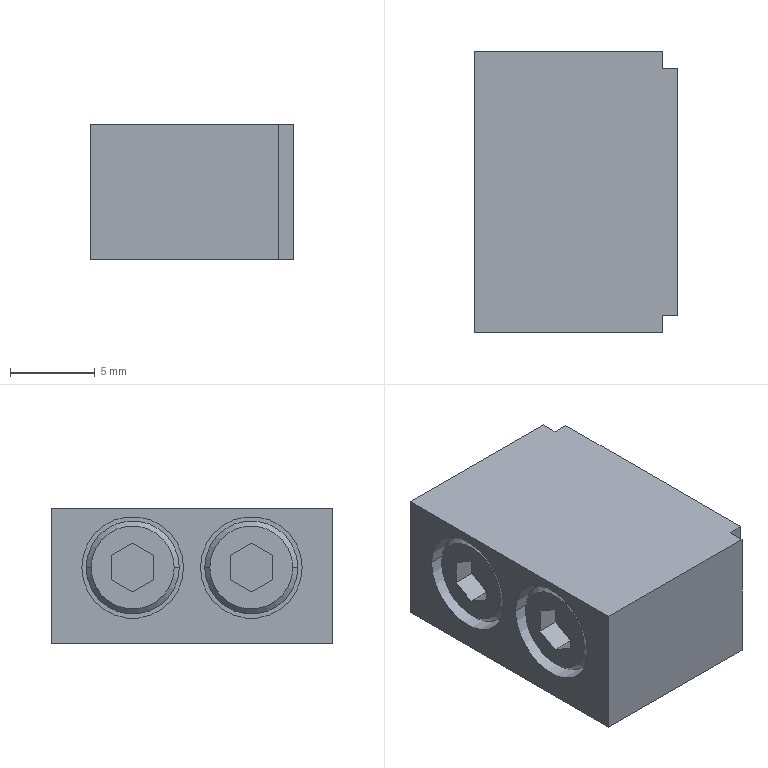Component | SolidWorks | MXQ8-30B-M9N_0_0_MXQ8-30B-M9N_0_0-2_MXQ8-30B-M9N_0_0_3_25-1 | 1 solid | 40 faces | box 12 x 16.6 x 8 mm | volume 1520 mm3 | plane 28 | cylinder 8 | cone 4 | commonest cylinder face diameters 6 x4 5.5 x4
STEP:
#1=COLOUR_RGB('',0.7922,0.8196,0.9333);
#2=FILL_AREA_STYLE_COLOUR('',#1);
#3=FILL_AREA_STYLE('',(#2));
#4=SURFACE_STYLE_FILL_AREA(#3);
#5=SURFACE_SIDE_STYLE('',(#4));
#6=SURFACE_STYLE_USAGE(.BOTH.,#5);
#7=PRESENTATION_STYLE_ASSIGNMENT((#6));
#8=CARTESIAN_POINT('',(0.7677,0.1496,1.417));
#9=VERTEX_POINT('',#8);
#10=CARTESIAN_POINT('',(0.7677,-0.08661,1.417));
#11=VERTEX_POINT('',#10);
#12=CARTESIAN_POINT('',(0.7677,0.0315,1.417));
#13=DIRECTION('',(-1.,0.,0.));
#14=DIRECTION('',(0.,-1.,0.));
#15=AXIS2_PLACEMENT_3D('',#12,#13,#14);
#16=CIRCLE('',#15,0.1181);
#17=EDGE_CURVE('',#9,#11,#16,.T.);
#18=ORIENTED_EDGE('',*,*,#17,.F.);
#19=CARTESIAN_POINT('',(0.6378,0.1496,1.417));
#20=VERTEX_POINT('',#19);
#21=CARTESIAN_POINT('',(0.6378,0.1496,1.417));
#22=DIRECTION('',(-1.,0.,0.));
#23=VECTOR('',#22,39.37);
#24=LINE('',#21,#23);
#25=EDGE_CURVE('',#9,#20,#24,.T.);
#26=ORIENTED_EDGE('',*,*,#25,.T.);
#27=CARTESIAN_POINT('',(0.6378,-0.08661,1.417));
#28=VERTEX_POINT('',#27);
#29=CARTESIAN_POINT('',(0.6378,0.0315,1.417));
#30=DIRECTION('',(1.,0.,0.));
#31=DIRECTION('',(0.,-1.,0.));
#32=AXIS2_PLACEMENT_3D('',#29,#30,#31);
#33=CIRCLE('',#32,0.1181);
#34=EDGE_CURVE('',#28,#20,#33,.T.);
#35=ORIENTED_EDGE('',*,*,#34,.F.);
#36=CARTESIAN_POINT('',(0.6378,-0.08661,1.417));
#37=DIRECTION('',(-1.,0.,0.));
#38=VECTOR('',#37,39.37);
#39=LINE('',#36,#38);
#40=EDGE_CURVE('',#11,#28,#39,.T.);
#41=ORIENTED_EDGE('',*,*,#40,.F.);
#42=EDGE_LOOP('',(#18,#26,#35,#41));
#43=FACE_OUTER_BOUND('',#42,.T.);
#44=CARTESIAN_POINT('',(0.6378,0.0315,1.417));
#45=DIRECTION('',(-1.,0.,0.));
#46=DIRECTION('',(0.,-1.,0.));
#47=AXIS2_PLACEMENT_3D('',#44,#45,#46);
#48=CYLINDRICAL_SURFACE('',#47,0.1181);
#49=ADVANCED_FACE('',(#43),#48,.F.);
#50=CARTESIAN_POINT('',(0.7677,0.4252,1.417));
#51=VERTEX_POINT('',#50);
#52=CARTESIAN_POINT('',(0.7677,0.189,1.417));
#53=VERTEX_POINT('',#52);
#54=CARTESIAN_POINT('',(0.7677,0.3071,1.417));
#55=DIRECTION('',(-1.,0.,0.));
#56=DIRECTION('',(0.,-1.,0.));
#57=AXIS2_PLACEMENT_3D('',#54,#55,#56);
#58=CIRCLE('',#57,0.1181);
#59=EDGE_CURVE('',#51,#53,#58,.T.);
#60=ORIENTED_EDGE('',*,*,#59,.F.);
#61=CARTESIAN_POINT('',(0.6378,0.4252,1.417));
#62=VERTEX_POINT('',#61);
#63=CARTESIAN_POINT('',(0.6378,0.4252,1.417));
#64=DIRECTION('',(-1.,0.,0.));
#65=VECTOR('',#64,39.37);
#66=LINE('',#63,#65);
#67=EDGE_CURVE('',#51,#62,#66,.T.);
#68=ORIENTED_EDGE('',*,*,#67,.T.);
#69=CARTESIAN_POINT('',(0.6378,0.189,1.417));
#70=VERTEX_POINT('',#69);
#71=CARTESIAN_POINT('',(0.6378,0.3071,1.417));
#72=DIRECTION('',(1.,0.,0.));
#73=DIRECTION('',(0.,-1.,0.));
#74=AXIS2_PLACEMENT_3D('',#71,#72,#73);
#75=CIRCLE('',#74,0.1181);
#76=EDGE_CURVE('',#70,#62,#75,.T.);
#77=ORIENTED_EDGE('',*,*,#76,.F.);
#78=CARTESIAN_POINT('',(0.6378,0.189,1.417));
#79=DIRECTION('',(-1.,0.,0.));
#80=VECTOR('',#79,39.37);
#81=LINE('',#78,#80);
#82=EDGE_CURVE('',#53,#70,#81,.T.);
#83=ORIENTED_EDGE('',*,*,#82,.F.);
#84=EDGE_LOOP('',(#60,#68,#77,#83));
#85=FACE_OUTER_BOUND('',#84,.T.);
#86=CARTESIAN_POINT('',(0.6378,0.3071,1.417));
#87=DIRECTION('',(-1.,0.,0.));
#88=DIRECTION('',(0.,-1.,0.));
#89=AXIS2_PLACEMENT_3D('',#86,#87,#88);
#90=CYLINDRICAL_SURFACE('',#89,0.1181);
#91=ADVANCED_FACE('',(#85),#90,.F.);
#92=CARTESIAN_POINT('',(0.6614,0.1398,1.417));
#93=VERTEX_POINT('',#92);
#94=CARTESIAN_POINT('',(0.6614,-0.07677,1.417));
#95=VERTEX_POINT('',#94);
#96=CARTESIAN_POINT('',(0.6614,0.0315,1.417));
#97=DIRECTION('',(1.,0.,0.));
#98=DIRECTION('',(0.,1.,0.));
#99=AXIS2_PLACEMENT_3D('',#96,#97,#98);
#100=CIRCLE('',#99,0.1083);
#101=EDGE_CURVE('',#93,#95,#100,.T.);
#102=ORIENTED_EDGE('',*,*,#101,.T.);
#103=CARTESIAN_POINT('',(0.7677,-0.07677,1.417));
#104=VERTEX_POINT('',#103);
#105=CARTESIAN_POINT('',(0.7146,-0.07677,1.417));
#106=DIRECTION('',(1.,0.,0.));
#107=VECTOR('',#106,39.37);
#108=LINE('',#105,#107);
#109=EDGE_CURVE('',#95,#104,#108,.T.);
#110=ORIENTED_EDGE('',*,*,#109,.T.);
#111=CARTESIAN_POINT('',(0.7677,0.1398,1.417));
#112=VERTEX_POINT('',#111);
#113=CARTESIAN_POINT('',(0.7677,0.0315,1.417));
#114=DIRECTION('',(1.,0.,0.));
#115=DIRECTION('',(0.,1.,0.));
#116=AXIS2_PLACEMENT_3D('',#113,#114,#115);
#117=CIRCLE('',#116,0.1083);
#118=EDGE_CURVE('',#112,#104,#117,.T.);
#119=ORIENTED_EDGE('',*,*,#118,.F.);
#120=CARTESIAN_POINT('',(0.7146,0.1398,1.417));
#121=DIRECTION('',(1.,0.,0.));
#122=VECTOR('',#121,39.37);
#123=LINE('',#120,#122);
#124=EDGE_CURVE('',#93,#112,#123,.T.);
#125=ORIENTED_EDGE('',*,*,#124,.F.);
#126=EDGE_LOOP('',(#102,#110,#119,#125));
#127=FACE_OUTER_BOUND('',#126,.T.);
#128=CARTESIAN_POINT('',(0.7146,0.0315,1.417));
#129=DIRECTION('',(1.,0.,0.));
#130=DIRECTION('',(0.,1.,0.));
#131=AXIS2_PLACEMENT_3D('',#128,#129,#130);
#132=CYLINDRICAL_SURFACE('',#131,0.1083);
#133=ADVANCED_FACE('',(#127),#132,.T.);
#134=CARTESIAN_POINT('',(0.6614,0.4154,1.417));
#135=VERTEX_POINT('',#134);
#136=CARTESIAN_POINT('',(0.6614,0.1988,1.417));
#137=VERTEX_POINT('',#136);
#138=CARTESIAN_POINT('',(0.6614,0.3071,1.417));
#139=DIRECTION('',(1.,0.,0.));
#140=DIRECTION('',(0.,1.,0.));
#141=AXIS2_PLACEMENT_3D('',#138,#139,#140);
#142=CIRCLE('',#141,0.1083);
#143=EDGE_CURVE('',#135,#137,#142,.T.);
#144=ORIENTED_EDGE('',*,*,#143,.T.);
#145=CARTESIAN_POINT('',(0.7677,0.1988,1.417));
#146=VERTEX_POINT('',#145);
#147=CARTESIAN_POINT('',(0.7146,0.1988,1.417));
#148=DIRECTION('',(1.,0.,0.));
#149=VECTOR('',#148,39.37);
#150=LINE('',#147,#149);
#151=EDGE_CURVE('',#137,#146,#150,.T.);
#152=ORIENTED_EDGE('',*,*,#151,.T.);
#153=CARTESIAN_POINT('',(0.7677,0.4154,1.417));
#154=VERTEX_POINT('',#153);
#155=CARTESIAN_POINT('',(0.7677,0.3071,1.417));
#156=DIRECTION('',(1.,0.,0.));
#157=DIRECTION('',(0.,1.,0.));
#158=AXIS2_PLACEMENT_3D('',#155,#156,#157);
#159=CIRCLE('',#158,0.1083);
#160=EDGE_CURVE('',#154,#146,#159,.T.);
#161=ORIENTED_EDGE('',*,*,#160,.F.);
#162=CARTESIAN_POINT('',(0.7146,0.4154,1.417));
#163=DIRECTION('',(1.,0.,0.));
#164=VECTOR('',#163,39.37);
#165=LINE('',#162,#164);
#166=EDGE_CURVE('',#135,#154,#165,.T.);
#167=ORIENTED_EDGE('',*,*,#166,.F.);
#168=EDGE_LOOP('',(#144,#152,#161,#167));
#169=FACE_OUTER_BOUND('',#168,.T.);
#170=CARTESIAN_POINT('',(0.7146,0.3071,1.417));
#171=DIRECTION('',(1.,0.,0.));
#172=DIRECTION('',(0.,1.,0.));
#173=AXIS2_PLACEMENT_3D('',#170,#171,#172);
#174=CYLINDRICAL_SURFACE('',#173,0.1083);
#175=ADVANCED_FACE('',(#169),#174,.T.);
#176=CARTESIAN_POINT('',(0.6496,0.128,1.417));
#177=VERTEX_POINT('',#176);
#178=CARTESIAN_POINT('',(0.6496,-0.06496,1.417));
#179=VERTEX_POINT('',#178);
#180=CARTESIAN_POINT('',(0.6496,0.0315,1.417));
#181=DIRECTION('',(1.,0.,0.));
#182=DIRECTION('',(0.,1.,0.));
#183=AXIS2_PLACEMENT_3D('',#180,#181,#182);
#184=CIRCLE('',#183,0.09646);
#185=EDGE_CURVE('',#177,#179,#184,.T.);
#186=ORIENTED_EDGE('',*,*,#185,.T.);
#187=CARTESIAN_POINT('',(0.6614,-0.07677,1.417));
#188=DIRECTION('',(0.7071,-0.7071,0.));
#189=VECTOR('',#188,39.37);
#190=LINE('',#187,#189);
#191=EDGE_CURVE('',#179,#95,#190,.T.);
#192=ORIENTED_EDGE('',*,*,#191,.T.);
#193=ORIENTED_EDGE('',*,*,#101,.F.);
#194=CARTESIAN_POINT('',(0.6614,0.1398,1.417));
#195=DIRECTION('',(0.7071,0.7071,0.));
#196=VECTOR('',#195,39.37);
#197=LINE('',#194,#196);
#198=EDGE_CURVE('',#177,#93,#197,.T.);
#199=ORIENTED_EDGE('',*,*,#198,.F.);
#200=EDGE_LOOP('',(#186,#192,#193,#199));
#201=FACE_OUTER_BOUND('',#200,.T.);
#202=CARTESIAN_POINT('',(0.6614,0.0315,1.417));
#203=DIRECTION('',(1.,0.,0.));
#204=DIRECTION('',(0.,1.,0.));
#205=AXIS2_PLACEMENT_3D('',#202,#203,#204);
#206=CONICAL_SURFACE('',#205,0.1083,0.7854);
#207=ADVANCED_FACE('',(#201),#206,.T.);
#208=CARTESIAN_POINT('',(0.6496,0.4035,1.417));
#209=VERTEX_POINT('',#208);
#210=CARTESIAN_POINT('',(0.6496,0.2106,1.417));
#211=VERTEX_POINT('',#210);
#212=CARTESIAN_POINT('',(0.6496,0.3071,1.417));
#213=DIRECTION('',(1.,0.,0.));
#214=DIRECTION('',(0.,1.,0.));
#215=AXIS2_PLACEMENT_3D('',#212,#213,#214);
#216=CIRCLE('',#215,0.09646);
#217=EDGE_CURVE('',#209,#211,#216,.T.);
#218=ORIENTED_EDGE('',*,*,#217,.T.);
#219=CARTESIAN_POINT('',(0.6614,0.1988,1.417));
#220=DIRECTION('',(0.7071,-0.7071,0.));
#221=VECTOR('',#220,39.37);
#222=LINE('',#219,#221);
#223=EDGE_CURVE('',#211,#137,#222,.T.);
#224=ORIENTED_EDGE('',*,*,#223,.T.);
#225=ORIENTED_EDGE('',*,*,#143,.F.);
#226=CARTESIAN_POINT('',(0.6614,0.4154,1.417));
#227=DIRECTION('',(0.7071,0.7071,0.));
#228=VECTOR('',#227,39.37);
#229=LINE('',#226,#228);
#230=EDGE_CURVE('',#209,#135,#229,.T.);
#231=ORIENTED_EDGE('',*,*,#230,.F.);
#232=EDGE_LOOP('',(#218,#224,#225,#231));
#233=FACE_OUTER_BOUND('',#232,.T.);
#234=CARTESIAN_POINT('',(0.6614,0.3071,1.417));
#235=DIRECTION('',(1.,0.,0.));
#236=DIRECTION('',(0.,1.,0.));
#237=AXIS2_PLACEMENT_3D('',#234,#235,#236);
#238=CONICAL_SURFACE('',#237,0.1083,0.7854);
#239=ADVANCED_FACE('',(#233),#238,.T.);
#240=CARTESIAN_POINT('',(0.6378,0.4961,1.555));
#241=VERTEX_POINT('',#240);
#242=CARTESIAN_POINT('',(1.075,0.4961,1.555));
#243=VERTEX_POINT('',#242);
#244=CARTESIAN_POINT('',(0.6378,0.4961,1.555));
#245=DIRECTION('',(1.,0.,0.));
#246=VECTOR('',#245,39.37);
#247=LINE('',#244,#246);
#248=EDGE_CURVE('',#241,#243,#247,.T.);
#249=ORIENTED_EDGE('',*,*,#248,.F.);
#250=CARTESIAN_POINT('',(0.6378,-0.1575,1.555));
#251=VERTEX_POINT('',#250);
#252=CARTESIAN_POINT('',(0.6378,-0.1575,1.555));
#253=DIRECTION('',(0.,1.,0.));
#254=VECTOR('',#253,39.37);
#255=LINE('',#252,#254);
#256=EDGE_CURVE('',#251,#241,#255,.T.);
#257=ORIENTED_EDGE('',*,*,#256,.F.);
#258=CARTESIAN_POINT('',(1.075,-0.1575,1.555));
#259=VERTEX_POINT('',#258);
#260=CARTESIAN_POINT('',(0.6378,-0.1575,1.555));
#261=DIRECTION('',(-1.,0.,0.));
#262=VECTOR('',#261,39.37);
#263=LINE('',#260,#262);
#264=EDGE_CURVE('',#259,#251,#263,.T.);
#265=ORIENTED_EDGE('',*,*,#264,.F.);
#266=CARTESIAN_POINT('',(1.075,-0.1181,1.555));
#267=VERTEX_POINT('',#266);
#268=CARTESIAN_POINT('',(1.075,-0.1181,1.555));
#269=DIRECTION('',(0.,1.,0.));
#270=VECTOR('',#269,39.37);
#271=LINE('',#268,#270);
#272=EDGE_CURVE('',#259,#267,#271,.T.);
#273=ORIENTED_EDGE('',*,*,#272,.T.);
#274=CARTESIAN_POINT('',(1.11,-0.1181,1.555));
#275=VERTEX_POINT('',#274);
#276=CARTESIAN_POINT('',(1.11,-0.1181,1.555));
#277=DIRECTION('',(1.,0.,0.));
#278=VECTOR('',#277,39.37);
#279=LINE('',#276,#278);
#280=EDGE_CURVE('',#267,#275,#279,.T.);
#281=ORIENTED_EDGE('',*,*,#280,.T.);
#282=CARTESIAN_POINT('',(1.11,0.4567,1.555));
#283=VERTEX_POINT('',#282);
#284=CARTESIAN_POINT('',(1.11,-0.1575,1.555));
#285=DIRECTION('',(0.,-1.,0.));
#286=VECTOR('',#285,39.37);
#287=LINE('',#284,#286);
#288=EDGE_CURVE('',#283,#275,#287,.T.);
#289=ORIENTED_EDGE('',*,*,#288,.F.);
#290=CARTESIAN_POINT('',(1.075,0.4567,1.555));
#291=VERTEX_POINT('',#290);
#292=CARTESIAN_POINT('',(1.075,0.4567,1.555));
#293=DIRECTION('',(-1.,0.,0.));
#294=VECTOR('',#293,39.37);
#295=LINE('',#292,#294);
#296=EDGE_CURVE('',#283,#291,#295,.T.);
#297=ORIENTED_EDGE('',*,*,#296,.T.);
#298=CARTESIAN_POINT('',(1.075,0.4961,1.555));
#299=DIRECTION('',(0.,1.,0.));
#300=VECTOR('',#299,39.37);
#301=LINE('',#298,#300);
#302=EDGE_CURVE('',#291,#243,#301,.T.);
#303=ORIENTED_EDGE('',*,*,#302,.T.);
#304=EDGE_LOOP('',(#249,#257,#265,#273,#281,#289,#297,#303));
#305=FACE_OUTER_BOUND('',#304,.T.);
#306=CARTESIAN_POINT('',(0.6378,-0.1575,1.555));
#307=DIRECTION('',(0.,0.,-1.));
#308=DIRECTION('',(0.,1.,0.));
#309=AXIS2_PLACEMENT_3D('',#306,#307,#308);
#310=PLANE('',#309);
#311=ADVANCED_FACE('',(#305),#310,.F.);
#312=CARTESIAN_POINT('',(0.6378,0.4961,1.24));
#313=VERTEX_POINT('',#312);
#314=CARTESIAN_POINT('',(0.6378,0.4961,1.555));
#315=DIRECTION('',(0.,0.,1.));
#316=VECTOR('',#315,39.37);
#317=LINE('',#314,#316);
#318=EDGE_CURVE('',#313,#241,#317,.T.);
#319=ORIENTED_EDGE('',*,*,#318,.T.);
#320=ORIENTED_EDGE('',*,*,#248,.T.);
#321=CARTESIAN_POINT('',(1.075,0.4961,1.24));
#322=VERTEX_POINT('',#321);
#323=CARTESIAN_POINT('',(1.075,0.4961,1.555));
#324=DIRECTION('',(0.,0.,-1.));
#325=VECTOR('',#324,39.37);
#326=LINE('',#323,#325);
#327=EDGE_CURVE('',#243,#322,#326,.T.);
#328=ORIENTED_EDGE('',*,*,#327,.T.);
#329=CARTESIAN_POINT('',(1.11,0.4961,1.24));
#330=DIRECTION('',(-1.,0.,0.));
#331=VECTOR('',#330,39.37);
#332=LINE('',#329,#331);
#333=EDGE_CURVE('',#322,#313,#332,.T.);
#334=ORIENTED_EDGE('',*,*,#333,.T.);
#335=EDGE_LOOP('',(#319,#320,#328,#334));
#336=FACE_OUTER_BOUND('',#335,.T.);
#337=CARTESIAN_POINT('',(1.11,0.4961,1.555));
#338=DIRECTION('',(0.,1.,0.));
#339=DIRECTION('',(-1.,0.,0.));
#340=AXIS2_PLACEMENT_3D('',#337,#338,#339);
#341=PLANE('',#340);
#342=ADVANCED_FACE('',(#336),#341,.T.);
#343=ORIENTED_EDGE('',*,*,#256,.T.);
#344=ORIENTED_EDGE('',*,*,#318,.F.);
#345=CARTESIAN_POINT('',(0.6378,-0.1575,1.24));
#346=VERTEX_POINT('',#345);
#347=CARTESIAN_POINT('',(0.6378,0.4961,1.24));
#348=DIRECTION('',(0.,-1.,0.));
#349=VECTOR('',#348,39.37);
#350=LINE('',#347,#349);
#351=EDGE_CURVE('',#313,#346,#350,.T.);
#352=ORIENTED_EDGE('',*,*,#351,.T.);
#353=CARTESIAN_POINT('',(0.6378,-0.1575,1.555));
#354=DIRECTION('',(0.,0.,1.));
#355=VECTOR('',#354,39.37);
#356=LINE('',#353,#355);
#357=EDGE_CURVE('',#346,#251,#356,.T.);
#358=ORIENTED_EDGE('',*,*,#357,.T.);
#359=EDGE_LOOP('',(#343,#344,#352,#358));
#360=FACE_OUTER_BOUND('',#359,.T.);
#361=ORIENTED_EDGE('',*,*,#34,.T.);
#362=CARTESIAN_POINT('',(0.6378,0.0315,1.417));
#363=DIRECTION('',(1.,0.,0.));
#364=DIRECTION('',(0.,-1.,0.));
#365=AXIS2_PLACEMENT_3D('',#362,#363,#364);
#366=CIRCLE('',#365,0.1181);
#367=EDGE_CURVE('',#20,#28,#366,.T.);
#368=ORIENTED_EDGE('',*,*,#367,.T.);
#369=EDGE_LOOP('',(#361,#368));
#370=FACE_BOUND('',#369,.T.);
#371=ORIENTED_EDGE('',*,*,#76,.T.);
#372=CARTESIAN_POINT('',(0.6378,0.3071,1.417));
#373=DIRECTION('',(1.,0.,0.));
#374=DIRECTION('',(0.,-1.,0.));
#375=AXIS2_PLACEMENT_3D('',#372,#373,#374);
#376=CIRCLE('',#375,0.1181);
#377=EDGE_CURVE('',#62,#70,#376,.T.);
#378=ORIENTED_EDGE('',*,*,#377,.T.);
#379=EDGE_LOOP('',(#371,#378));
#380=FACE_BOUND('',#379,.T.);
#381=CARTESIAN_POINT('',(0.6378,0.4961,1.555));
#382=DIRECTION('',(-1.,0.,0.));
#383=DIRECTION('',(0.,-1.,0.));
#384=AXIS2_PLACEMENT_3D('',#381,#382,#383);
#385=PLANE('',#384);
#386=ADVANCED_FACE('',(#360,#370,#380),#385,.T.);
#387=ORIENTED_EDGE('',*,*,#357,.F.);
#388=CARTESIAN_POINT('',(1.075,-0.1575,1.24));
#389=VERTEX_POINT('',#388);
#390=CARTESIAN_POINT('',(0.6378,-0.1575,1.24));
#391=DIRECTION('',(1.,0.,0.));
#392=VECTOR('',#391,39.37);
#393=LINE('',#390,#392);
#394=EDGE_CURVE('',#346,#389,#393,.T.);
#395=ORIENTED_EDGE('',*,*,#394,.T.);
#396=CARTESIAN_POINT('',(1.075,-0.1575,1.555));
#397=DIRECTION('',(0.,0.,1.));
#398=VECTOR('',#397,39.37);
#399=LINE('',#396,#398);
#400=EDGE_CURVE('',#389,#259,#399,.T.);
#401=ORIENTED_EDGE('',*,*,#400,.T.);
#402=ORIENTED_EDGE('',*,*,#264,.T.);
#403=EDGE_LOOP('',(#387,#395,#401,#402));
#404=FACE_OUTER_BOUND('',#403,.T.);
#405=CARTESIAN_POINT('',(0.6378,-0.1575,1.555));
#406=DIRECTION('',(0.,-1.,0.));
#407=DIRECTION('',(1.,0.,0.));
#408=AXIS2_PLACEMENT_3D('',#405,#406,#407);
#409=PLANE('',#408);
#410=ADVANCED_FACE('',(#404),#409,.T.);
#411=CARTESIAN_POINT('',(1.11,-0.1181,1.24));
#412=VERTEX_POINT('',#411);
#413=CARTESIAN_POINT('',(1.11,-0.1181,1.555));
#414=DIRECTION('',(0.,0.,-1.));
#415=VECTOR('',#414,39.37);
#416=LINE('',#413,#415);
#417=EDGE_CURVE('',#275,#412,#416,.T.);
#418=ORIENTED_EDGE('',*,*,#417,.T.);
#419=CARTESIAN_POINT('',(1.11,0.4567,1.24));
#420=VERTEX_POINT('',#419);
#421=CARTESIAN_POINT('',(1.11,-0.1575,1.24));
#422=DIRECTION('',(0.,1.,0.));
#423=VECTOR('',#422,39.37);
#424=LINE('',#421,#423);
#425=EDGE_CURVE('',#412,#420,#424,.T.);
#426=ORIENTED_EDGE('',*,*,#425,.T.);
#427=CARTESIAN_POINT('',(1.11,0.4567,1.555));
#428=DIRECTION('',(0.,0.,1.));
#429=VECTOR('',#428,39.37);
#430=LINE('',#427,#429);
#431=EDGE_CURVE('',#420,#283,#430,.T.);
#432=ORIENTED_EDGE('',*,*,#431,.T.);
#433=ORIENTED_EDGE('',*,*,#288,.T.);
#434=EDGE_LOOP('',(#418,#426,#432,#433));
#435=FACE_OUTER_BOUND('',#434,.T.);
#436=CARTESIAN_POINT('',(1.11,-0.1575,1.555));
#437=DIRECTION('',(1.,0.,0.));
#438=DIRECTION('',(0.,1.,0.));
#439=AXIS2_PLACEMENT_3D('',#436,#437,#438);
#440=PLANE('',#439);
#441=ADVANCED_FACE('',(#435),#440,.T.);
#442=ORIENTED_EDGE('',*,*,#351,.F.);
#443=ORIENTED_EDGE('',*,*,#333,.F.);
#444=CARTESIAN_POINT('',(1.075,0.4567,1.24));
#445=VERTEX_POINT('',#444);
#446=CARTESIAN_POINT('',(1.075,-0.1575,1.24));
#447=DIRECTION('',(0.,-1.,0.));
#448=VECTOR('',#447,39.37);
#449=LINE('',#446,#448);
#450=EDGE_CURVE('',#322,#445,#449,.T.);
#451=ORIENTED_EDGE('',*,*,#450,.T.);
#452=CARTESIAN_POINT('',(0.6378,0.4567,1.24));
#453=DIRECTION('',(1.,0.,0.));
#454=VECTOR('',#453,39.37);
#455=LINE('',#452,#454);
#456=EDGE_CURVE('',#445,#420,#455,.T.);
#457=ORIENTED_EDGE('',*,*,#456,.T.);
#458=ORIENTED_EDGE('',*,*,#425,.F.);
#459=CARTESIAN_POINT('',(1.075,-0.1181,1.24));
#460=VERTEX_POINT('',#459);
#461=CARTESIAN_POINT('',(0.6378,-0.1181,1.24));
#462=DIRECTION('',(-1.,0.,0.));
#463=VECTOR('',#462,39.37);
#464=LINE('',#461,#463);
#465=EDGE_CURVE('',#412,#460,#464,.T.);
#466=ORIENTED_EDGE('',*,*,#465,.T.);
#467=CARTESIAN_POINT('',(1.075,-0.1575,1.24));
#468=DIRECTION('',(0.,-1.,0.));
#469=VECTOR('',#468,39.37);
#470=LINE('',#467,#469);
#471=EDGE_CURVE('',#460,#389,#470,.T.);
#472=ORIENTED_EDGE('',*,*,#471,.T.);
#473=ORIENTED_EDGE('',*,*,#394,.F.);
#474=EDGE_LOOP('',(#442,#443,#451,#457,#458,#466,#472,#473));
#475=FACE_OUTER_BOUND('',#474,.T.);
#476=CARTESIAN_POINT('',(0.6378,-0.1575,1.24));
#477=DIRECTION('',(0.,0.,-1.));
#478=DIRECTION('',(0.,1.,0.));
#479=AXIS2_PLACEMENT_3D('',#476,#477,#478);
#480=PLANE('',#479);
#481=ADVANCED_FACE('',(#475),#480,.T.);
#482=ORIENTED_EDGE('',*,*,#327,.F.);
#483=ORIENTED_EDGE('',*,*,#302,.F.);
#484=CARTESIAN_POINT('',(1.075,0.4567,1.555));
#485=DIRECTION('',(0.,0.,1.));
#486=VECTOR('',#485,39.37);
#487=LINE('',#484,#486);
#488=EDGE_CURVE('',#445,#291,#487,.T.);
#489=ORIENTED_EDGE('',*,*,#488,.F.);
#490=ORIENTED_EDGE('',*,*,#450,.F.);
#491=EDGE_LOOP('',(#482,#483,#489,#490));
#492=FACE_OUTER_BOUND('',#491,.T.);
#493=CARTESIAN_POINT('',(1.075,0.4961,1.555));
#494=DIRECTION('',(-1.,0.,0.));
#495=DIRECTION('',(0.,-1.,0.));
#496=AXIS2_PLACEMENT_3D('',#493,#494,#495);
#497=PLANE('',#496);
#498=ADVANCED_FACE('',(#492),#497,.F.);
#499=ORIENTED_EDGE('',*,*,#25,.F.);
#500=CARTESIAN_POINT('',(0.7677,0.0315,1.417));
#501=DIRECTION('',(-1.,0.,0.));
#502=DIRECTION('',(0.,-1.,0.));
#503=AXIS2_PLACEMENT_3D('',#500,#501,#502);
#504=CIRCLE('',#503,0.1181);
#505=EDGE_CURVE('',#11,#9,#504,.T.);
#506=ORIENTED_EDGE('',*,*,#505,.F.);
#507=ORIENTED_EDGE('',*,*,#40,.T.);
#508=ORIENTED_EDGE('',*,*,#367,.F.);
#509=EDGE_LOOP('',(#499,#506,#507,#508));
#510=FACE_OUTER_BOUND('',#509,.T.);
#511=CARTESIAN_POINT('',(0.6378,0.0315,1.417));
#512=DIRECTION('',(-1.,0.,0.));
#513=DIRECTION('',(0.,-1.,0.));
#514=AXIS2_PLACEMENT_3D('',#511,#512,#513);
#515=CYLINDRICAL_SURFACE('',#514,0.1181);
#516=ADVANCED_FACE('',(#510),#515,.F.);
#517=ORIENTED_EDGE('',*,*,#67,.F.);
#518=CARTESIAN_POINT('',(0.7677,0.3071,1.417));
#519=DIRECTION('',(-1.,0.,0.));
#520=DIRECTION('',(0.,-1.,0.));
#521=AXIS2_PLACEMENT_3D('',#518,#519,#520);
#522=CIRCLE('',#521,0.1181);
#523=EDGE_CURVE('',#53,#51,#522,.T.);
#524=ORIENTED_EDGE('',*,*,#523,.F.);
#525=ORIENTED_EDGE('',*,*,#82,.T.);
#526=ORIENTED_EDGE('',*,*,#377,.F.);
#527=EDGE_LOOP('',(#517,#524,#525,#526));
#528=FACE_OUTER_BOUND('',#527,.T.);
#529=CARTESIAN_POINT('',(0.6378,0.3071,1.417));
#530=DIRECTION('',(-1.,0.,0.));
#531=DIRECTION('',(0.,-1.,0.));
#532=AXIS2_PLACEMENT_3D('',#529,#530,#531);
#533=CYLINDRICAL_SURFACE('',#532,0.1181);
#534=ADVANCED_FACE('',(#528),#533,.F.);
#535=CARTESIAN_POINT('',(1.075,-0.1181,1.555));
#536=DIRECTION('',(0.,0.,-1.));
#537=VECTOR('',#536,39.37);
#538=LINE('',#535,#537);
#539=EDGE_CURVE('',#267,#460,#538,.T.);
#540=ORIENTED_EDGE('',*,*,#539,.F.);
#541=ORIENTED_EDGE('',*,*,#272,.F.);
#542=ORIENTED_EDGE('',*,*,#400,.F.);
#543=ORIENTED_EDGE('',*,*,#471,.F.);
#544=EDGE_LOOP('',(#540,#541,#542,#543));
#545=FACE_OUTER_BOUND('',#544,.T.);
#546=CARTESIAN_POINT('',(1.075,-0.1181,1.555));
#547=DIRECTION('',(-1.,0.,0.));
#548=DIRECTION('',(0.,-1.,0.));
#549=AXIS2_PLACEMENT_3D('',#546,#547,#548);
#550=PLANE('',#549);
#551=ADVANCED_FACE('',(#545),#550,.F.);
#552=ORIENTED_EDGE('',*,*,#417,.F.);
#553=ORIENTED_EDGE('',*,*,#280,.F.);
#554=ORIENTED_EDGE('',*,*,#539,.T.);
#555=ORIENTED_EDGE('',*,*,#465,.F.);
#556=EDGE_LOOP('',(#552,#553,#554,#555));
#557=FACE_OUTER_BOUND('',#556,.T.);
#558=CARTESIAN_POINT('',(1.11,-0.1181,1.555));
#559=DIRECTION('',(0.,1.,0.));
#560=DIRECTION('',(-1.,0.,0.));
#561=AXIS2_PLACEMENT_3D('',#558,#559,#560);
#562=PLANE('',#561);
#563=ADVANCED_FACE('',(#557),#562,.F.);
#564=ORIENTED_EDGE('',*,*,#488,.T.);
#565=ORIENTED_EDGE('',*,*,#296,.F.);
#566=ORIENTED_EDGE('',*,*,#431,.F.);
#567=ORIENTED_EDGE('',*,*,#456,.F.);
#568=EDGE_LOOP('',(#564,#565,#566,#567));
#569=FACE_OUTER_BOUND('',#568,.T.);
#570=CARTESIAN_POINT('',(1.075,0.4567,1.555));
#571=DIRECTION('',(0.,-1.,0.));
#572=DIRECTION('',(1.,0.,0.));
#573=AXIS2_PLACEMENT_3D('',#570,#571,#572);
#574=PLANE('',#573);
#575=ADVANCED_FACE('',(#569),#574,.F.);
#576=ORIENTED_EDGE('',*,*,#505,.T.);
#577=ORIENTED_EDGE('',*,*,#17,.T.);
#578=EDGE_LOOP('',(#576,#577));
#579=FACE_OUTER_BOUND('',#578,.T.);
#580=ORIENTED_EDGE('',*,*,#118,.T.);
#581=CARTESIAN_POINT('',(0.7677,0.0315,1.417));
#582=DIRECTION('',(1.,0.,0.));
#583=DIRECTION('',(0.,1.,0.));
#584=AXIS2_PLACEMENT_3D('',#581,#582,#583);
#585=CIRCLE('',#584,0.1083);
#586=EDGE_CURVE('',#104,#112,#585,.T.);
#587=ORIENTED_EDGE('',*,*,#586,.T.);
#588=EDGE_LOOP('',(#580,#587));
#589=FACE_BOUND('',#588,.T.);
#590=CARTESIAN_POINT('',(0.7677,-0.1575,1.555));
#591=DIRECTION('',(-1.,0.,0.));
#592=DIRECTION('',(0.,-1.,0.));
#593=AXIS2_PLACEMENT_3D('',#590,#591,#592);
#594=PLANE('',#593);
#595=ADVANCED_FACE('',(#579,#589),#594,.T.);
#596=ORIENTED_EDGE('',*,*,#523,.T.);
#597=ORIENTED_EDGE('',*,*,#59,.T.);
#598=EDGE_LOOP('',(#596,#597));
#599=FACE_OUTER_BOUND('',#598,.T.);
#600=ORIENTED_EDGE('',*,*,#160,.T.);
#601=CARTESIAN_POINT('',(0.7677,0.3071,1.417));
#602=DIRECTION('',(1.,0.,0.));
#603=DIRECTION('',(0.,1.,0.));
#604=AXIS2_PLACEMENT_3D('',#601,#602,#603);
#605=CIRCLE('',#604,0.1083);
#606=EDGE_CURVE('',#146,#154,#605,.T.);
#607=ORIENTED_EDGE('',*,*,#606,.T.);
#608=EDGE_LOOP('',(#600,#607));
#609=FACE_BOUND('',#608,.T.);
#610=CARTESIAN_POINT('',(0.7677,-0.1575,1.555));
#611=DIRECTION('',(-1.,0.,0.));
#612=DIRECTION('',(0.,-1.,0.));
#613=AXIS2_PLACEMENT_3D('',#610,#611,#612);
#614=PLANE('',#613);
#615=ADVANCED_FACE('',(#599,#609),#614,.T.);
#616=ORIENTED_EDGE('',*,*,#109,.F.);
#617=CARTESIAN_POINT('',(0.6614,0.0315,1.417));
#618=DIRECTION('',(1.,0.,0.));
#619=DIRECTION('',(0.,1.,0.));
#620=AXIS2_PLACEMENT_3D('',#617,#618,#619);
#621=CIRCLE('',#620,0.1083);
#622=EDGE_CURVE('',#95,#93,#621,.T.);
#623=ORIENTED_EDGE('',*,*,#622,.T.);
#624=ORIENTED_EDGE('',*,*,#124,.T.);
#625=ORIENTED_EDGE('',*,*,#586,.F.);
#626=EDGE_LOOP('',(#616,#623,#624,#625));
#627=FACE_OUTER_BOUND('',#626,.T.);
#628=CARTESIAN_POINT('',(0.7146,0.0315,1.417));
#629=DIRECTION('',(1.,0.,0.));
#630=DIRECTION('',(0.,1.,0.));
#631=AXIS2_PLACEMENT_3D('',#628,#629,#630);
#632=CYLINDRICAL_SURFACE('',#631,0.1083);
#633=ADVANCED_FACE('',(#627),#632,.T.);
#634=ORIENTED_EDGE('',*,*,#151,.F.);
#635=CARTESIAN_POINT('',(0.6614,0.3071,1.417));
#636=DIRECTION('',(1.,0.,0.));
#637=DIRECTION('',(0.,1.,0.));
#638=AXIS2_PLACEMENT_3D('',#635,#636,#637);
#639=CIRCLE('',#638,0.1083);
#640=EDGE_CURVE('',#137,#135,#639,.T.);
#641=ORIENTED_EDGE('',*,*,#640,.T.);
#642=ORIENTED_EDGE('',*,*,#166,.T.);
#643=ORIENTED_EDGE('',*,*,#606,.F.);
#644=EDGE_LOOP('',(#634,#641,#642,#643));
#645=FACE_OUTER_BOUND('',#644,.T.);
#646=CARTESIAN_POINT('',(0.7146,0.3071,1.417));
#647=DIRECTION('',(1.,0.,0.));
#648=DIRECTION('',(0.,1.,0.));
#649=AXIS2_PLACEMENT_3D('',#646,#647,#648);
#650=CYLINDRICAL_SURFACE('',#649,0.1083);
#651=ADVANCED_FACE('',(#645),#650,.T.);
#652=ORIENTED_EDGE('',*,*,#191,.F.);
#653=CARTESIAN_POINT('',(0.6496,0.0315,1.417));
#654=DIRECTION('',(1.,0.,0.));
#655=DIRECTION('',(0.,1.,0.));
#656=AXIS2_PLACEMENT_3D('',#653,#654,#655);
#657=CIRCLE('',#656,0.09646);
#658=EDGE_CURVE('',#179,#177,#657,.T.);
#659=ORIENTED_EDGE('',*,*,#658,.T.);
#660=ORIENTED_EDGE('',*,*,#198,.T.);
#661=ORIENTED_EDGE('',*,*,#622,.F.);
#662=EDGE_LOOP('',(#652,#659,#660,#661));
#663=FACE_OUTER_BOUND('',#662,.T.);
#664=CARTESIAN_POINT('',(0.6614,0.0315,1.417));
#665=DIRECTION('',(1.,0.,0.));
#666=DIRECTION('',(0.,1.,0.));
#667=AXIS2_PLACEMENT_3D('',#664,#665,#666);
#668=CONICAL_SURFACE('',#667,0.1083,0.7854);
#669=ADVANCED_FACE('',(#663),#668,.T.);
#670=ORIENTED_EDGE('',*,*,#223,.F.);
#671=CARTESIAN_POINT('',(0.6496,0.3071,1.417));
#672=DIRECTION('',(1.,0.,0.));
#673=DIRECTION('',(0.,1.,0.));
#674=AXIS2_PLACEMENT_3D('',#671,#672,#673);
#675=CIRCLE('',#674,0.09646);
#676=EDGE_CURVE('',#211,#209,#675,.T.);
#677=ORIENTED_EDGE('',*,*,#676,.T.);
#678=ORIENTED_EDGE('',*,*,#230,.T.);
#679=ORIENTED_EDGE('',*,*,#640,.F.);
#680=EDGE_LOOP('',(#670,#677,#678,#679));
#681=FACE_OUTER_BOUND('',#680,.T.);
#682=CARTESIAN_POINT('',(0.6614,0.3071,1.417));
#683=DIRECTION('',(1.,0.,0.));
#684=DIRECTION('',(0.,1.,0.));
#685=AXIS2_PLACEMENT_3D('',#682,#683,#684);
#686=CONICAL_SURFACE('',#685,0.1083,0.7854);
#687=ADVANCED_FACE('',(#681),#686,.T.);
#688=ORIENTED_EDGE('',*,*,#185,.F.);
#689=ORIENTED_EDGE('',*,*,#658,.F.);
#690=EDGE_LOOP('',(#688,#689));
#691=FACE_OUTER_BOUND('',#690,.T.);
#692=CARTESIAN_POINT('',(0.6496,0.0315,1.36));
#693=VERTEX_POINT('',#692);
#694=CARTESIAN_POINT('',(0.6496,0.08071,1.389));
#695=VERTEX_POINT('',#694);
#696=CARTESIAN_POINT('',(0.6496,0.0315,1.36));
#697=DIRECTION('',(0.,0.866,0.5));
#698=VECTOR('',#697,39.37);
#699=LINE('',#696,#698);
#700=EDGE_CURVE('',#693,#695,#699,.T.);
#701=ORIENTED_EDGE('',*,*,#700,.T.);
#702=CARTESIAN_POINT('',(0.6496,0.08071,1.446));
#703=VERTEX_POINT('',#702);
#704=CARTESIAN_POINT('',(0.6496,0.08071,1.369));
#705=DIRECTION('',(0.,0.,1.));
#706=VECTOR('',#705,39.37);
#707=LINE('',#704,#706);
#708=EDGE_CURVE('',#695,#703,#707,.T.);
#709=ORIENTED_EDGE('',*,*,#708,.T.);
#710=CARTESIAN_POINT('',(0.6496,0.0315,1.474));
#711=VERTEX_POINT('',#710);
#712=CARTESIAN_POINT('',(0.6496,0.08071,1.446));
#713=DIRECTION('',(0.,-0.866,0.5));
#714=VECTOR('',#713,39.37);
#715=LINE('',#712,#714);
#716=EDGE_CURVE('',#703,#711,#715,.T.);
#717=ORIENTED_EDGE('',*,*,#716,.T.);
#718=CARTESIAN_POINT('',(0.6496,-0.01772,1.446));
#719=VERTEX_POINT('',#718);
#720=CARTESIAN_POINT('',(0.6496,0.0315,1.474));
#721=DIRECTION('',(0.,-0.866,-0.5));
#722=VECTOR('',#721,39.37);
#723=LINE('',#720,#722);
#724=EDGE_CURVE('',#711,#719,#723,.T.);
#725=ORIENTED_EDGE('',*,*,#724,.T.);
#726=CARTESIAN_POINT('',(0.6496,-0.01772,1.389));
#727=VERTEX_POINT('',#726);
#728=CARTESIAN_POINT('',(0.6496,-0.01772,1.369));
#729=DIRECTION('',(0.,0.,-1.));
#730=VECTOR('',#729,39.37);
#731=LINE('',#728,#730);
#732=EDGE_CURVE('',#719,#727,#731,.T.);
#733=ORIENTED_EDGE('',*,*,#732,.T.);
#734=CARTESIAN_POINT('',(0.6496,-0.01772,1.389));
#735=DIRECTION('',(0.,0.866,-0.5));
#736=VECTOR('',#735,39.37);
#737=LINE('',#734,#736);
#738=EDGE_CURVE('',#727,#693,#737,.T.);
#739=ORIENTED_EDGE('',*,*,#738,.T.);
#740=EDGE_LOOP('',(#701,#709,#717,#725,#733,#739));
#741=FACE_BOUND('',#740,.T.);
#742=CARTESIAN_POINT('',(0.6496,0.0315,1.369));
#743=DIRECTION('',(-1.,0.,0.));
#744=DIRECTION('',(0.,-1.,0.));
#745=AXIS2_PLACEMENT_3D('',#742,#743,#744);
#746=PLANE('',#745);
#747=ADVANCED_FACE('',(#691,#741),#746,.T.);
#748=ORIENTED_EDGE('',*,*,#217,.F.);
#749=ORIENTED_EDGE('',*,*,#676,.F.);
#750=EDGE_LOOP('',(#748,#749));
#751=FACE_OUTER_BOUND('',#750,.T.);
#752=CARTESIAN_POINT('',(0.6496,0.3563,1.389));
#753=VERTEX_POINT('',#752);
#754=CARTESIAN_POINT('',(0.6496,0.3563,1.446));
#755=VERTEX_POINT('',#754);
#756=CARTESIAN_POINT('',(0.6496,0.3563,1.369));
#757=DIRECTION('',(0.,0.,1.));
#758=VECTOR('',#757,39.37);
#759=LINE('',#756,#758);
#760=EDGE_CURVE('',#753,#755,#759,.T.);
#761=ORIENTED_EDGE('',*,*,#760,.T.);
#762=CARTESIAN_POINT('',(0.6496,0.3071,1.474));
#763=VERTEX_POINT('',#762);
#764=CARTESIAN_POINT('',(0.6496,0.3563,1.446));
#765=DIRECTION('',(0.,-0.866,0.5));
#766=VECTOR('',#765,39.37);
#767=LINE('',#764,#766);
#768=EDGE_CURVE('',#755,#763,#767,.T.);
#769=ORIENTED_EDGE('',*,*,#768,.T.);
#770=CARTESIAN_POINT('',(0.6496,0.2579,1.446));
#771=VERTEX_POINT('',#770);
#772=CARTESIAN_POINT('',(0.6496,0.3071,1.474));
#773=DIRECTION('',(0.,-0.866,-0.5));
#774=VECTOR('',#773,39.37);
#775=LINE('',#772,#774);
#776=EDGE_CURVE('',#763,#771,#775,.T.);
#777=ORIENTED_EDGE('',*,*,#776,.T.);
#778=CARTESIAN_POINT('',(0.6496,0.2579,1.389));
#779=VERTEX_POINT('',#778);
#780=CARTESIAN_POINT('',(0.6496,0.2579,1.369));
#781=DIRECTION('',(0.,0.,-1.));
#782=VECTOR('',#781,39.37);
#783=LINE('',#780,#782);
#784=EDGE_CURVE('',#771,#779,#783,.T.);
#785=ORIENTED_EDGE('',*,*,#784,.T.);
#786=CARTESIAN_POINT('',(0.6496,0.3071,1.36));
#787=VERTEX_POINT('',#786);
#788=CARTESIAN_POINT('',(0.6496,0.2579,1.389));
#789=DIRECTION('',(0.,0.866,-0.5));
#790=VECTOR('',#789,39.37);
#791=LINE('',#788,#790);
#792=EDGE_CURVE('',#779,#787,#791,.T.);
#793=ORIENTED_EDGE('',*,*,#792,.T.);
#794=CARTESIAN_POINT('',(0.6496,0.3071,1.36));
#795=DIRECTION('',(0.,0.866,0.5));
#796=VECTOR('',#795,39.37);
#797=LINE('',#794,#796);
#798=EDGE_CURVE('',#787,#753,#797,.T.);
#799=ORIENTED_EDGE('',*,*,#798,.T.);
#800=EDGE_LOOP('',(#761,#769,#777,#785,#793,#799));
#801=FACE_BOUND('',#800,.T.);
#802=CARTESIAN_POINT('',(0.6496,0.3071,1.369));
#803=DIRECTION('',(-1.,0.,0.));
#804=DIRECTION('',(0.,-1.,0.));
#805=AXIS2_PLACEMENT_3D('',#802,#803,#804);
#806=PLANE('',#805);
#807=ADVANCED_FACE('',(#751,#801),#806,.T.);
#808=CARTESIAN_POINT('',(0.7008,0.08071,1.446));
#809=VERTEX_POINT('',#808);
#810=CARTESIAN_POINT('',(0.6496,0.08071,1.446));
#811=DIRECTION('',(1.,0.,0.));
#812=VECTOR('',#811,39.37);
#813=LINE('',#810,#812);
#814=EDGE_CURVE('',#703,#809,#813,.T.);
#815=ORIENTED_EDGE('',*,*,#814,.F.);
#816=ORIENTED_EDGE('',*,*,#708,.F.);
#817=CARTESIAN_POINT('',(0.7008,0.08071,1.389));
#818=VERTEX_POINT('',#817);
#819=CARTESIAN_POINT('',(0.6496,0.08071,1.389));
#820=DIRECTION('',(-1.,0.,0.));
#821=VECTOR('',#820,39.37);
#822=LINE('',#819,#821);
#823=EDGE_CURVE('',#818,#695,#822,.T.);
#824=ORIENTED_EDGE('',*,*,#823,.F.);
#825=CARTESIAN_POINT('',(0.7008,0.08071,1.446));
#826=DIRECTION('',(0.,0.,-1.));
#827=VECTOR('',#826,39.37);
#828=LINE('',#825,#827);
#829=EDGE_CURVE('',#809,#818,#828,.T.);
#830=ORIENTED_EDGE('',*,*,#829,.F.);
#831=EDGE_LOOP('',(#815,#816,#824,#830));
#832=FACE_OUTER_BOUND('',#831,.T.);
#833=CARTESIAN_POINT('',(0.6496,0.08071,1.446));
#834=DIRECTION('',(0.,1.,0.));
#835=DIRECTION('',(-1.,0.,0.));
#836=AXIS2_PLACEMENT_3D('',#833,#834,#835);
#837=PLANE('',#836);
#838=ADVANCED_FACE('',(#832),#837,.F.);
#839=ORIENTED_EDGE('',*,*,#823,.T.);
#840=ORIENTED_EDGE('',*,*,#700,.F.);
#841=CARTESIAN_POINT('',(0.7008,0.0315,1.36));
#842=VERTEX_POINT('',#841);
#843=CARTESIAN_POINT('',(0.6496,0.0315,1.36));
#844=DIRECTION('',(-1.,0.,0.));
#845=VECTOR('',#844,39.37);
#846=LINE('',#843,#845);
#847=EDGE_CURVE('',#842,#693,#846,.T.);
#848=ORIENTED_EDGE('',*,*,#847,.F.);
#849=CARTESIAN_POINT('',(0.7008,0.08071,1.389));
#850=DIRECTION('',(0.,-0.866,-0.5));
#851=VECTOR('',#850,39.37);
#852=LINE('',#849,#851);
#853=EDGE_CURVE('',#818,#842,#852,.T.);
#854=ORIENTED_EDGE('',*,*,#853,.F.);
#855=EDGE_LOOP('',(#839,#840,#848,#854));
#856=FACE_OUTER_BOUND('',#855,.T.);
#857=CARTESIAN_POINT('',(0.6496,0.08071,1.389));
#858=DIRECTION('',(0.,0.5,-0.866));
#859=DIRECTION('',(0.,0.866,0.5));
#860=AXIS2_PLACEMENT_3D('',#857,#858,#859);
#861=PLANE('',#860);
#862=ADVANCED_FACE('',(#856),#861,.F.);
#863=ORIENTED_EDGE('',*,*,#847,.T.);
#864=ORIENTED_EDGE('',*,*,#738,.F.);
#865=CARTESIAN_POINT('',(0.7008,-0.01772,1.389));
#866=VERTEX_POINT('',#865);
#867=CARTESIAN_POINT('',(0.6496,-0.01772,1.389));
#868=DIRECTION('',(-1.,0.,0.));
#869=VECTOR('',#868,39.37);
#870=LINE('',#867,#869);
#871=EDGE_CURVE('',#866,#727,#870,.T.);
#872=ORIENTED_EDGE('',*,*,#871,.F.);
#873=CARTESIAN_POINT('',(0.7008,0.0315,1.36));
#874=DIRECTION('',(0.,-0.866,0.5));
#875=VECTOR('',#874,39.37);
#876=LINE('',#873,#875);
#877=EDGE_CURVE('',#842,#866,#876,.T.);
#878=ORIENTED_EDGE('',*,*,#877,.F.);
#879=EDGE_LOOP('',(#863,#864,#872,#878));
#880=FACE_OUTER_BOUND('',#879,.T.);
#881=CARTESIAN_POINT('',(0.6496,0.0315,1.36));
#882=DIRECTION('',(0.,-0.5,-0.866));
#883=DIRECTION('',(0.,0.866,-0.5));
#884=AXIS2_PLACEMENT_3D('',#881,#882,#883);
#885=PLANE('',#884);
#886=ADVANCED_FACE('',(#880),#885,.F.);
#887=ORIENTED_EDGE('',*,*,#871,.T.);
#888=ORIENTED_EDGE('',*,*,#732,.F.);
#889=CARTESIAN_POINT('',(0.7008,-0.01772,1.446));
#890=VERTEX_POINT('',#889);
#891=CARTESIAN_POINT('',(0.6496,-0.01772,1.446));
#892=DIRECTION('',(-1.,0.,0.));
#893=VECTOR('',#892,39.37);
#894=LINE('',#891,#893);
#895=EDGE_CURVE('',#890,#719,#894,.T.);
#896=ORIENTED_EDGE('',*,*,#895,.F.);
#897=CARTESIAN_POINT('',(0.7008,-0.01772,1.389));
#898=DIRECTION('',(0.,0.,1.));
#899=VECTOR('',#898,39.37);
#900=LINE('',#897,#899);
#901=EDGE_CURVE('',#866,#890,#900,.T.);
#902=ORIENTED_EDGE('',*,*,#901,.F.);
#903=EDGE_LOOP('',(#887,#888,#896,#902));
#904=FACE_OUTER_BOUND('',#903,.T.);
#905=CARTESIAN_POINT('',(0.6496,-0.01772,1.389));
#906=DIRECTION('',(0.,-1.,0.));
#907=DIRECTION('',(1.,0.,0.));
#908=AXIS2_PLACEMENT_3D('',#905,#906,#907);
#909=PLANE('',#908);
#910=ADVANCED_FACE('',(#904),#909,.F.);
#911=ORIENTED_EDGE('',*,*,#895,.T.);
#912=ORIENTED_EDGE('',*,*,#724,.F.);
#913=CARTESIAN_POINT('',(0.7008,0.0315,1.474));
#914=VERTEX_POINT('',#913);
#915=CARTESIAN_POINT('',(0.6496,0.0315,1.474));
#916=DIRECTION('',(-1.,0.,0.));
#917=VECTOR('',#916,39.37);
#918=LINE('',#915,#917);
#919=EDGE_CURVE('',#914,#711,#918,.T.);
#920=ORIENTED_EDGE('',*,*,#919,.F.);
#921=CARTESIAN_POINT('',(0.7008,-0.01772,1.446));
#922=DIRECTION('',(0.,0.866,0.5));
#923=VECTOR('',#922,39.37);
#924=LINE('',#921,#923);
#925=EDGE_CURVE('',#890,#914,#924,.T.);
#926=ORIENTED_EDGE('',*,*,#925,.F.);
#927=EDGE_LOOP('',(#911,#912,#920,#926));
#928=FACE_OUTER_BOUND('',#927,.T.);
#929=CARTESIAN_POINT('',(0.6496,-0.01772,1.446));
#930=DIRECTION('',(0.,-0.5,0.866));
#931=DIRECTION('',(0.,-0.866,-0.5));
#932=AXIS2_PLACEMENT_3D('',#929,#930,#931);
#933=PLANE('',#932);
#934=ADVANCED_FACE('',(#928),#933,.F.);
#935=ORIENTED_EDGE('',*,*,#919,.T.);
#936=ORIENTED_EDGE('',*,*,#716,.F.);
#937=ORIENTED_EDGE('',*,*,#814,.T.);
#938=CARTESIAN_POINT('',(0.7008,0.0315,1.474));
#939=DIRECTION('',(0.,0.866,-0.5));
#940=VECTOR('',#939,39.37);
#941=LINE('',#938,#940);
#942=EDGE_CURVE('',#914,#809,#941,.T.);
#943=ORIENTED_EDGE('',*,*,#942,.F.);
#944=EDGE_LOOP('',(#935,#936,#937,#943));
#945=FACE_OUTER_BOUND('',#944,.T.);
#946=CARTESIAN_POINT('',(0.6496,0.0315,1.474));
#947=DIRECTION('',(0.,0.5,0.866));
#948=DIRECTION('',(0.,-0.866,0.5));
#949=AXIS2_PLACEMENT_3D('',#946,#947,#948);
#950=PLANE('',#949);
#951=ADVANCED_FACE('',(#945),#950,.F.);
#952=CARTESIAN_POINT('',(0.7008,0.3071,1.474));
#953=VERTEX_POINT('',#952);
#954=CARTESIAN_POINT('',(0.6496,0.3071,1.474));
#955=DIRECTION('',(1.,0.,0.));
#956=VECTOR('',#955,39.37);
#957=LINE('',#954,#956);
#958=EDGE_CURVE('',#763,#953,#957,.T.);
#959=ORIENTED_EDGE('',*,*,#958,.F.);
#960=ORIENTED_EDGE('',*,*,#768,.F.);
#961=CARTESIAN_POINT('',(0.7008,0.3563,1.446));
#962=VERTEX_POINT('',#961);
#963=CARTESIAN_POINT('',(0.6496,0.3563,1.446));
#964=DIRECTION('',(-1.,0.,0.));
#965=VECTOR('',#964,39.37);
#966=LINE('',#963,#965);
#967=EDGE_CURVE('',#962,#755,#966,.T.);
#968=ORIENTED_EDGE('',*,*,#967,.F.);
#969=CARTESIAN_POINT('',(0.7008,0.3071,1.474));
#970=DIRECTION('',(0.,0.866,-0.5));
#971=VECTOR('',#970,39.37);
#972=LINE('',#969,#971);
#973=EDGE_CURVE('',#953,#962,#972,.T.);
#974=ORIENTED_EDGE('',*,*,#973,.F.);
#975=EDGE_LOOP('',(#959,#960,#968,#974));
#976=FACE_OUTER_BOUND('',#975,.T.);
#977=CARTESIAN_POINT('',(0.6496,0.3071,1.474));
#978=DIRECTION('',(0.,0.5,0.866));
#979=DIRECTION('',(0.,-0.866,0.5));
#980=AXIS2_PLACEMENT_3D('',#977,#978,#979);
#981=PLANE('',#980);
#982=ADVANCED_FACE('',(#976),#981,.F.);
#983=ORIENTED_EDGE('',*,*,#967,.T.);
#984=ORIENTED_EDGE('',*,*,#760,.F.);
#985=CARTESIAN_POINT('',(0.7008,0.3563,1.389));
#986=VERTEX_POINT('',#985);
#987=CARTESIAN_POINT('',(0.6496,0.3563,1.389));
#988=DIRECTION('',(-1.,0.,0.));
#989=VECTOR('',#988,39.37);
#990=LINE('',#987,#989);
#991=EDGE_CURVE('',#986,#753,#990,.T.);
#992=ORIENTED_EDGE('',*,*,#991,.F.);
#993=CARTESIAN_POINT('',(0.7008,0.3563,1.446));
#994=DIRECTION('',(0.,0.,-1.));
#995=VECTOR('',#994,39.37);
#996=LINE('',#993,#995);
#997=EDGE_CURVE('',#962,#986,#996,.T.);
#998=ORIENTED_EDGE('',*,*,#997,.F.);
#999=EDGE_LOOP('',(#983,#984,#992,#998));
#1000=FACE_OUTER_BOUND('',#999,.T.);
#1001=CARTESIAN_POINT('',(0.6496,0.3563,1.446));
#1002=DIRECTION('',(0.,1.,0.));
#1003=DIRECTION('',(-1.,0.,0.));
#1004=AXIS2_PLACEMENT_3D('',#1001,#1002,#1003);
#1005=PLANE('',#1004);
#1006=ADVANCED_FACE('',(#1000),#1005,.F.);
#1007=ORIENTED_EDGE('',*,*,#991,.T.);
#1008=ORIENTED_EDGE('',*,*,#798,.F.);
#1009=CARTESIAN_POINT('',(0.7008,0.3071,1.36));
#1010=VERTEX_POINT('',#1009);
#1011=CARTESIAN_POINT('',(0.6496,0.3071,1.36));
#1012=DIRECTION('',(-1.,0.,0.));
#1013=VECTOR('',#1012,39.37);
#1014=LINE('',#1011,#1013);
#1015=EDGE_CURVE('',#1010,#787,#1014,.T.);
#1016=ORIENTED_EDGE('',*,*,#1015,.F.);
#1017=CARTESIAN_POINT('',(0.7008,0.3563,1.389));
#1018=DIRECTION('',(0.,-0.866,-0.5));
#1019=VECTOR('',#1018,39.37);
#1020=LINE('',#1017,#1019);
#1021=EDGE_CURVE('',#986,#1010,#1020,.T.);
#1022=ORIENTED_EDGE('',*,*,#1021,.F.);
#1023=EDGE_LOOP('',(#1007,#1008,#1016,#1022));
#1024=FACE_OUTER_BOUND('',#1023,.T.);
#1025=CARTESIAN_POINT('',(0.6496,0.3563,1.389));
#1026=DIRECTION('',(0.,0.5,-0.866));
#1027=DIRECTION('',(0.,0.866,0.5));
#1028=AXIS2_PLACEMENT_3D('',#1025,#1026,#1027);
#1029=PLANE('',#1028);
#1030=ADVANCED_FACE('',(#1024),#1029,.F.);
#1031=ORIENTED_EDGE('',*,*,#1015,.T.);
#1032=ORIENTED_EDGE('',*,*,#792,.F.);
#1033=CARTESIAN_POINT('',(0.7008,0.2579,1.389));
#1034=VERTEX_POINT('',#1033);
#1035=CARTESIAN_POINT('',(0.6496,0.2579,1.389));
#1036=DIRECTION('',(-1.,0.,0.));
#1037=VECTOR('',#1036,39.37);
#1038=LINE('',#1035,#1037);
#1039=EDGE_CURVE('',#1034,#779,#1038,.T.);
#1040=ORIENTED_EDGE('',*,*,#1039,.F.);
#1041=CARTESIAN_POINT('',(0.7008,0.3071,1.36));
#1042=DIRECTION('',(0.,-0.866,0.5));
#1043=VECTOR('',#1042,39.37);
#1044=LINE('',#1041,#1043);
#1045=EDGE_CURVE('',#1010,#1034,#1044,.T.);
#1046=ORIENTED_EDGE('',*,*,#1045,.F.);
#1047=EDGE_LOOP('',(#1031,#1032,#1040,#1046));
#1048=FACE_OUTER_BOUND('',#1047,.T.);
#1049=CARTESIAN_POINT('',(0.6496,0.3071,1.36));
#1050=DIRECTION('',(0.,-0.5,-0.866));
#1051=DIRECTION('',(0.,0.866,-0.5));
#1052=AXIS2_PLACEMENT_3D('',#1049,#1050,#1051);
#1053=PLANE('',#1052);
#1054=ADVANCED_FACE('',(#1048),#1053,.F.);
#1055=ORIENTED_EDGE('',*,*,#1039,.T.);
#1056=ORIENTED_EDGE('',*,*,#784,.F.);
#1057=CARTESIAN_POINT('',(0.7008,0.2579,1.446));
#1058=VERTEX_POINT('',#1057);
#1059=CARTESIAN_POINT('',(0.6496,0.2579,1.446));
#1060=DIRECTION('',(-1.,0.,0.));
#1061=VECTOR('',#1060,39.37);
#1062=LINE('',#1059,#1061);
#1063=EDGE_CURVE('',#1058,#771,#1062,.T.);
#1064=ORIENTED_EDGE('',*,*,#1063,.F.);
#1065=CARTESIAN_POINT('',(0.7008,0.2579,1.389));
#1066=DIRECTION('',(0.,0.,1.));
#1067=VECTOR('',#1066,39.37);
#1068=LINE('',#1065,#1067);
#1069=EDGE_CURVE('',#1034,#1058,#1068,.T.);
#1070=ORIENTED_EDGE('',*,*,#1069,.F.);
#1071=EDGE_LOOP('',(#1055,#1056,#1064,#1070));
#1072=FACE_OUTER_BOUND('',#1071,.T.);
#1073=CARTESIAN_POINT('',(0.6496,0.2579,1.389));
#1074=DIRECTION('',(0.,-1.,0.));
#1075=DIRECTION('',(1.,0.,0.));
#1076=AXIS2_PLACEMENT_3D('',#1073,#1074,#1075);
#1077=PLANE('',#1076);
#1078=ADVANCED_FACE('',(#1072),#1077,.F.);
#1079=ORIENTED_EDGE('',*,*,#1063,.T.);
#1080=ORIENTED_EDGE('',*,*,#776,.F.);
#1081=ORIENTED_EDGE('',*,*,#958,.T.);
#1082=CARTESIAN_POINT('',(0.7008,0.2579,1.446));
#1083=DIRECTION('',(0.,0.866,0.5));
#1084=VECTOR('',#1083,39.37);
#1085=LINE('',#1082,#1084);
#1086=EDGE_CURVE('',#1058,#953,#1085,.T.);
#1087=ORIENTED_EDGE('',*,*,#1086,.F.);
#1088=EDGE_LOOP('',(#1079,#1080,#1081,#1087));
#1089=FACE_OUTER_BOUND('',#1088,.T.);
#1090=CARTESIAN_POINT('',(0.6496,0.2579,1.446));
#1091=DIRECTION('',(0.,-0.5,0.866));
#1092=DIRECTION('',(0.,-0.866,-0.5));
#1093=AXIS2_PLACEMENT_3D('',#1090,#1091,#1092);
#1094=PLANE('',#1093);
#1095=ADVANCED_FACE('',(#1089),#1094,.F.);
#1096=ORIENTED_EDGE('',*,*,#901,.T.);
#1097=ORIENTED_EDGE('',*,*,#925,.T.);
#1098=ORIENTED_EDGE('',*,*,#942,.T.);
#1099=ORIENTED_EDGE('',*,*,#829,.T.);
#1100=ORIENTED_EDGE('',*,*,#853,.T.);
#1101=ORIENTED_EDGE('',*,*,#877,.T.);
#1102=EDGE_LOOP('',(#1096,#1097,#1098,#1099,#1100,#1101));
#1103=FACE_OUTER_BOUND('',#1102,.T.);
#1104=CARTESIAN_POINT('',(0.7008,-0.1575,1.555));
#1105=DIRECTION('',(-1.,0.,0.));
#1106=DIRECTION('',(0.,-1.,0.));
#1107=AXIS2_PLACEMENT_3D('',#1104,#1105,#1106);
#1108=PLANE('',#1107);
#1109=ADVANCED_FACE('',(#1103),#1108,.T.);
#1110=ORIENTED_EDGE('',*,*,#1045,.T.);
#1111=ORIENTED_EDGE('',*,*,#1069,.T.);
#1112=ORIENTED_EDGE('',*,*,#1086,.T.);
#1113=ORIENTED_EDGE('',*,*,#973,.T.);
#1114=ORIENTED_EDGE('',*,*,#997,.T.);
#1115=ORIENTED_EDGE('',*,*,#1021,.T.);
#1116=EDGE_LOOP('',(#1110,#1111,#1112,#1113,#1114,#1115));
#1117=FACE_OUTER_BOUND('',#1116,.T.);
#1118=CARTESIAN_POINT('',(0.7008,-0.1575,1.555));
#1119=DIRECTION('',(-1.,0.,0.));
#1120=DIRECTION('',(0.,-1.,0.));
#1121=AXIS2_PLACEMENT_3D('',#1118,#1119,#1120);
#1122=PLANE('',#1121);
#1123=ADVANCED_FACE('',(#1117),#1122,.T.);
#1124=CLOSED_SHELL('',(#49,#91,#133,#175,#207,#239,#311,#342,#386,#410,#441,#481,#498,#516,#534,#551,#563,#575,#595,#615,#633,#651,#669,#687,#747,#807,#838,#862,#886,#910,#934,#951,#982,#1006,#1030,#1054,#1078,#1095,#1109,#1123));
#1125=MANIFOLD_SOLID_BREP('',#1124);
#1126=STYLED_ITEM('',(#7),#1125);
#1127=PRESENTATION_LAYER_ASSIGNMENT('','',(#1126));
#1128=CARTESIAN_POINT('',(0.,0.,0.));
#1129=DIRECTION('',(0.,0.,1.));
#1130=DIRECTION('',(1.,0.,0.));
#1131=AXIS2_PLACEMENT_3D('',#1128,#1129,#1130);
#1132=(LENGTH_UNIT()NAMED_UNIT(*)SI_UNIT($,.METRE.));
#1133=LENGTH_MEASURE_WITH_UNIT(LENGTH_MEASURE(0.0254),#1132);
#1134=DIMENSIONAL_EXPONENTS(1.,0.,0.,0.,0.,0.,0.);
#1135=(CONVERSION_BASED_UNIT('',#1133)LENGTH_UNIT()NAMED_UNIT(#1134));
#1136=UNCERTAINTY_MEASURE_WITH_UNIT(LENGTH_MEASURE(0.00001),#1135,'','');
#1137=(NAMED_UNIT(*)PLANE_ANGLE_UNIT()SI_UNIT($,.RADIAN.));
#1138=(NAMED_UNIT(*)SI_UNIT($,.STERADIAN.)SOLID_ANGLE_UNIT());
#1139=(GEOMETRIC_REPRESENTATION_CONTEXT(3)GLOBAL_UNCERTAINTY_ASSIGNED_CONTEXT((#1136))GLOBAL_UNIT_ASSIGNED_CONTEXT((#1135,#1137,#1138))REPRESENTATION_CONTEXT('',''));
#1140=ADVANCED_BREP_SHAPE_REPRESENTATION('',(#1125,#1131),#1139);
#1141=(LENGTH_UNIT()NAMED_UNIT(*)SI_UNIT($,.METRE.));
#1142=LENGTH_MEASURE_WITH_UNIT(LENGTH_MEASURE(0.0254),#1141);
#1143=DIMENSIONAL_EXPONENTS(1.,0.,0.,0.,0.,0.,0.);
#1144=(CONVERSION_BASED_UNIT('',#1142)LENGTH_UNIT()NAMED_UNIT(#1143));
#1145=UNCERTAINTY_MEASURE_WITH_UNIT(LENGTH_MEASURE(0.00001),#1144,'','');
#1146=(NAMED_UNIT(*)PLANE_ANGLE_UNIT()SI_UNIT($,.RADIAN.));
#1147=(NAMED_UNIT(*)SI_UNIT($,.STERADIAN.)SOLID_ANGLE_UNIT());
#1148=(GEOMETRIC_REPRESENTATION_CONTEXT(3)GLOBAL_UNCERTAINTY_ASSIGNED_CONTEXT((#1145))GLOBAL_UNIT_ASSIGNED_CONTEXT((#1144,#1146,#1147))REPRESENTATION_CONTEXT('',''));
#1149=MECHANICAL_DESIGN_GEOMETRIC_PRESENTATION_REPRESENTATION('',(#1126),#1148);